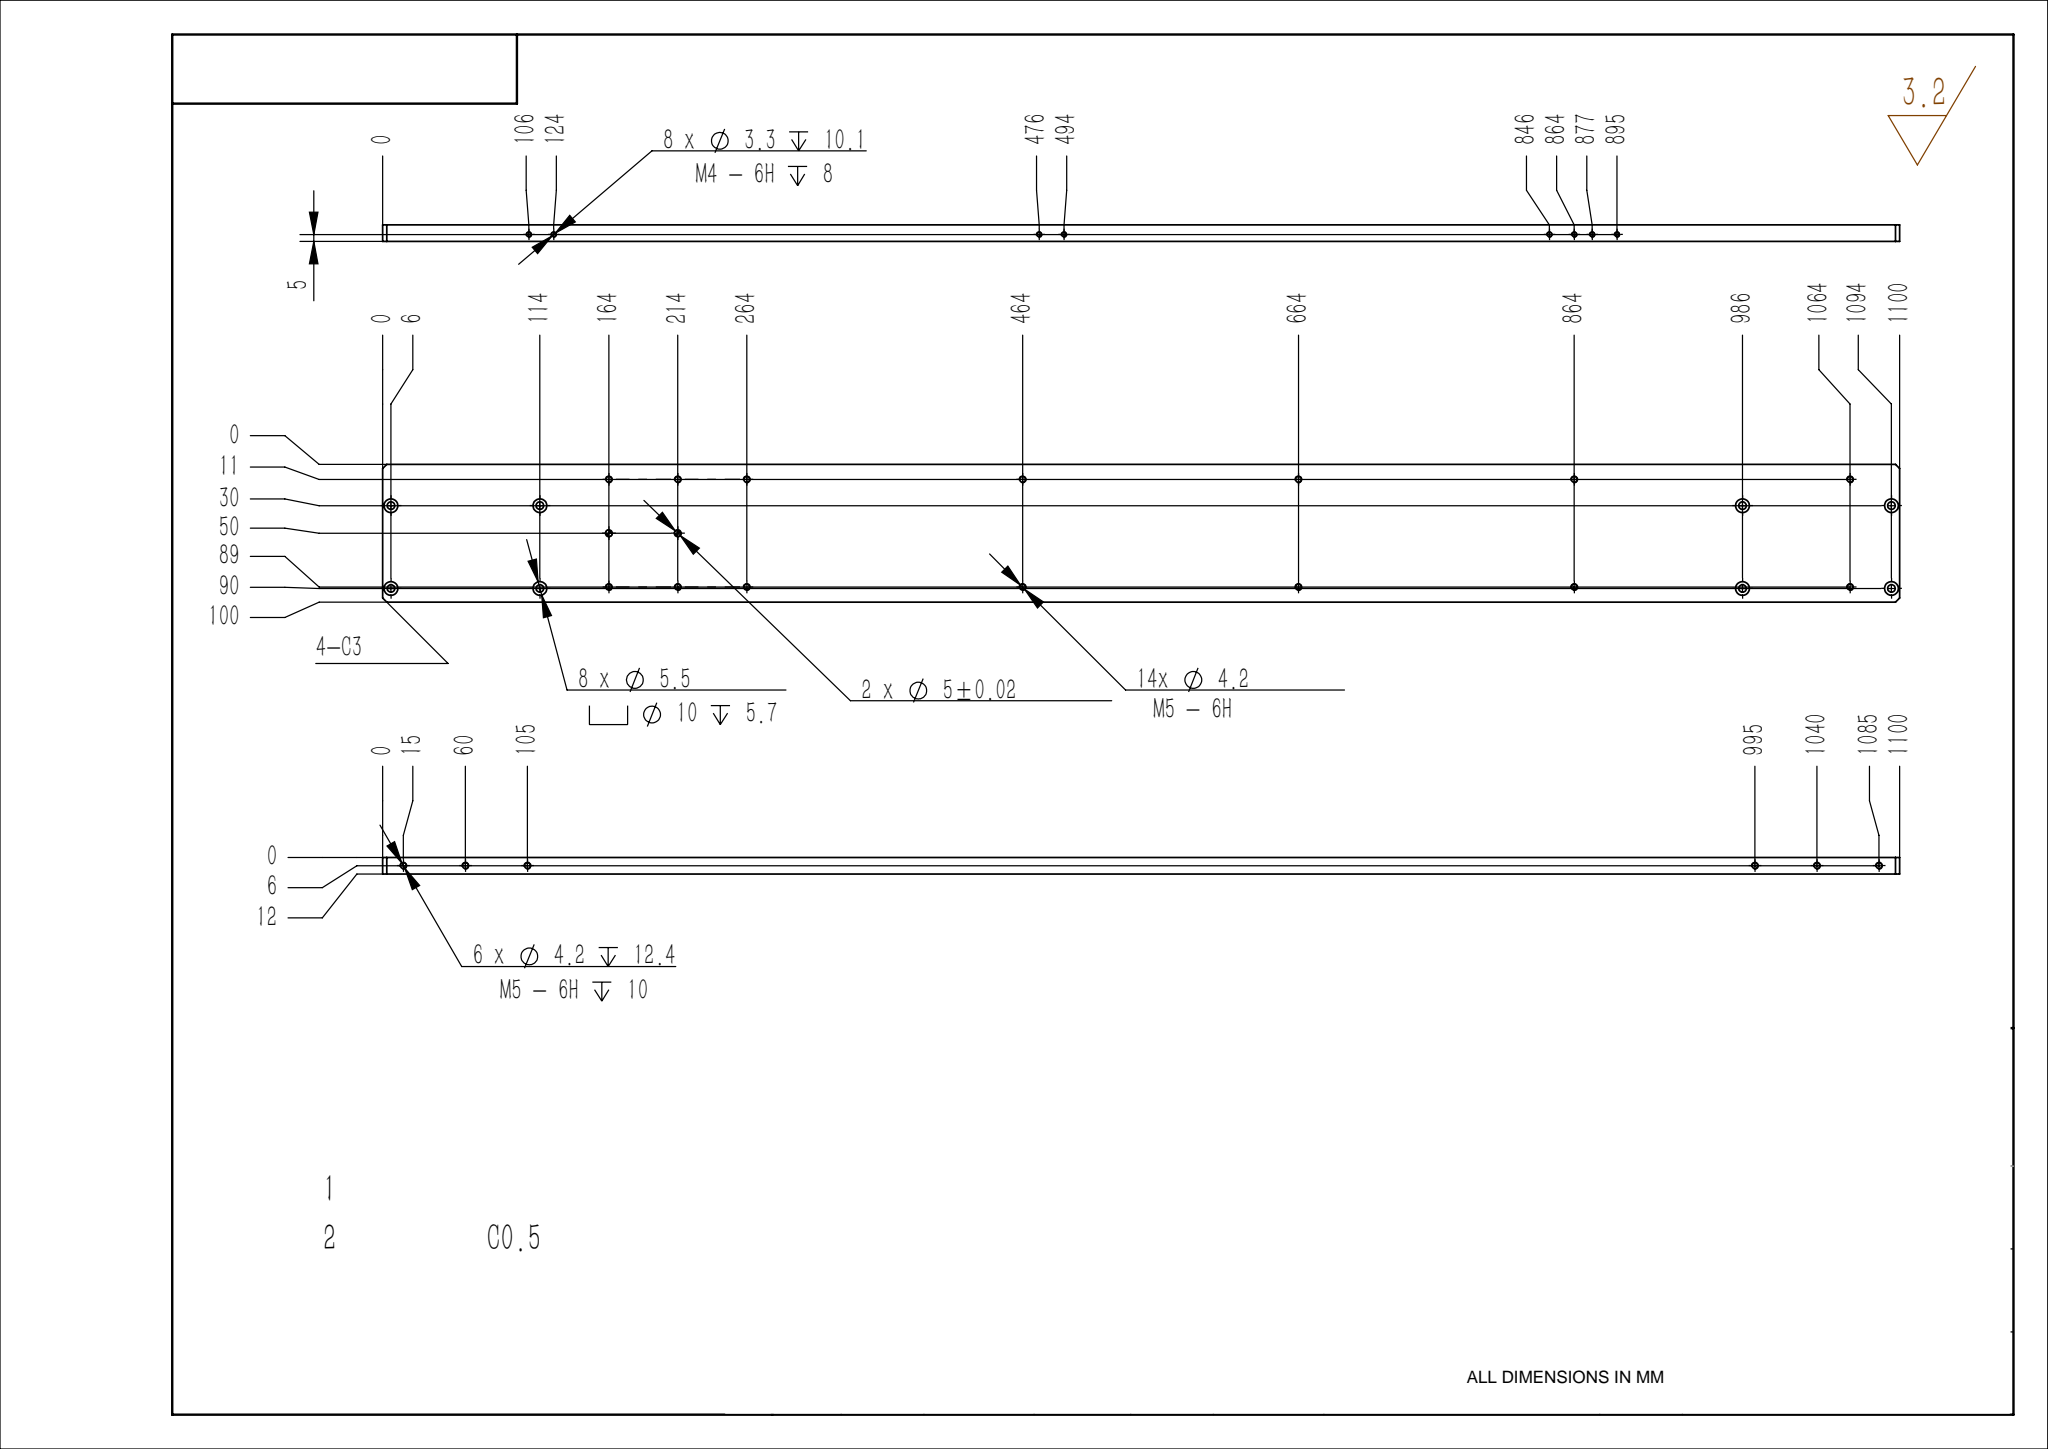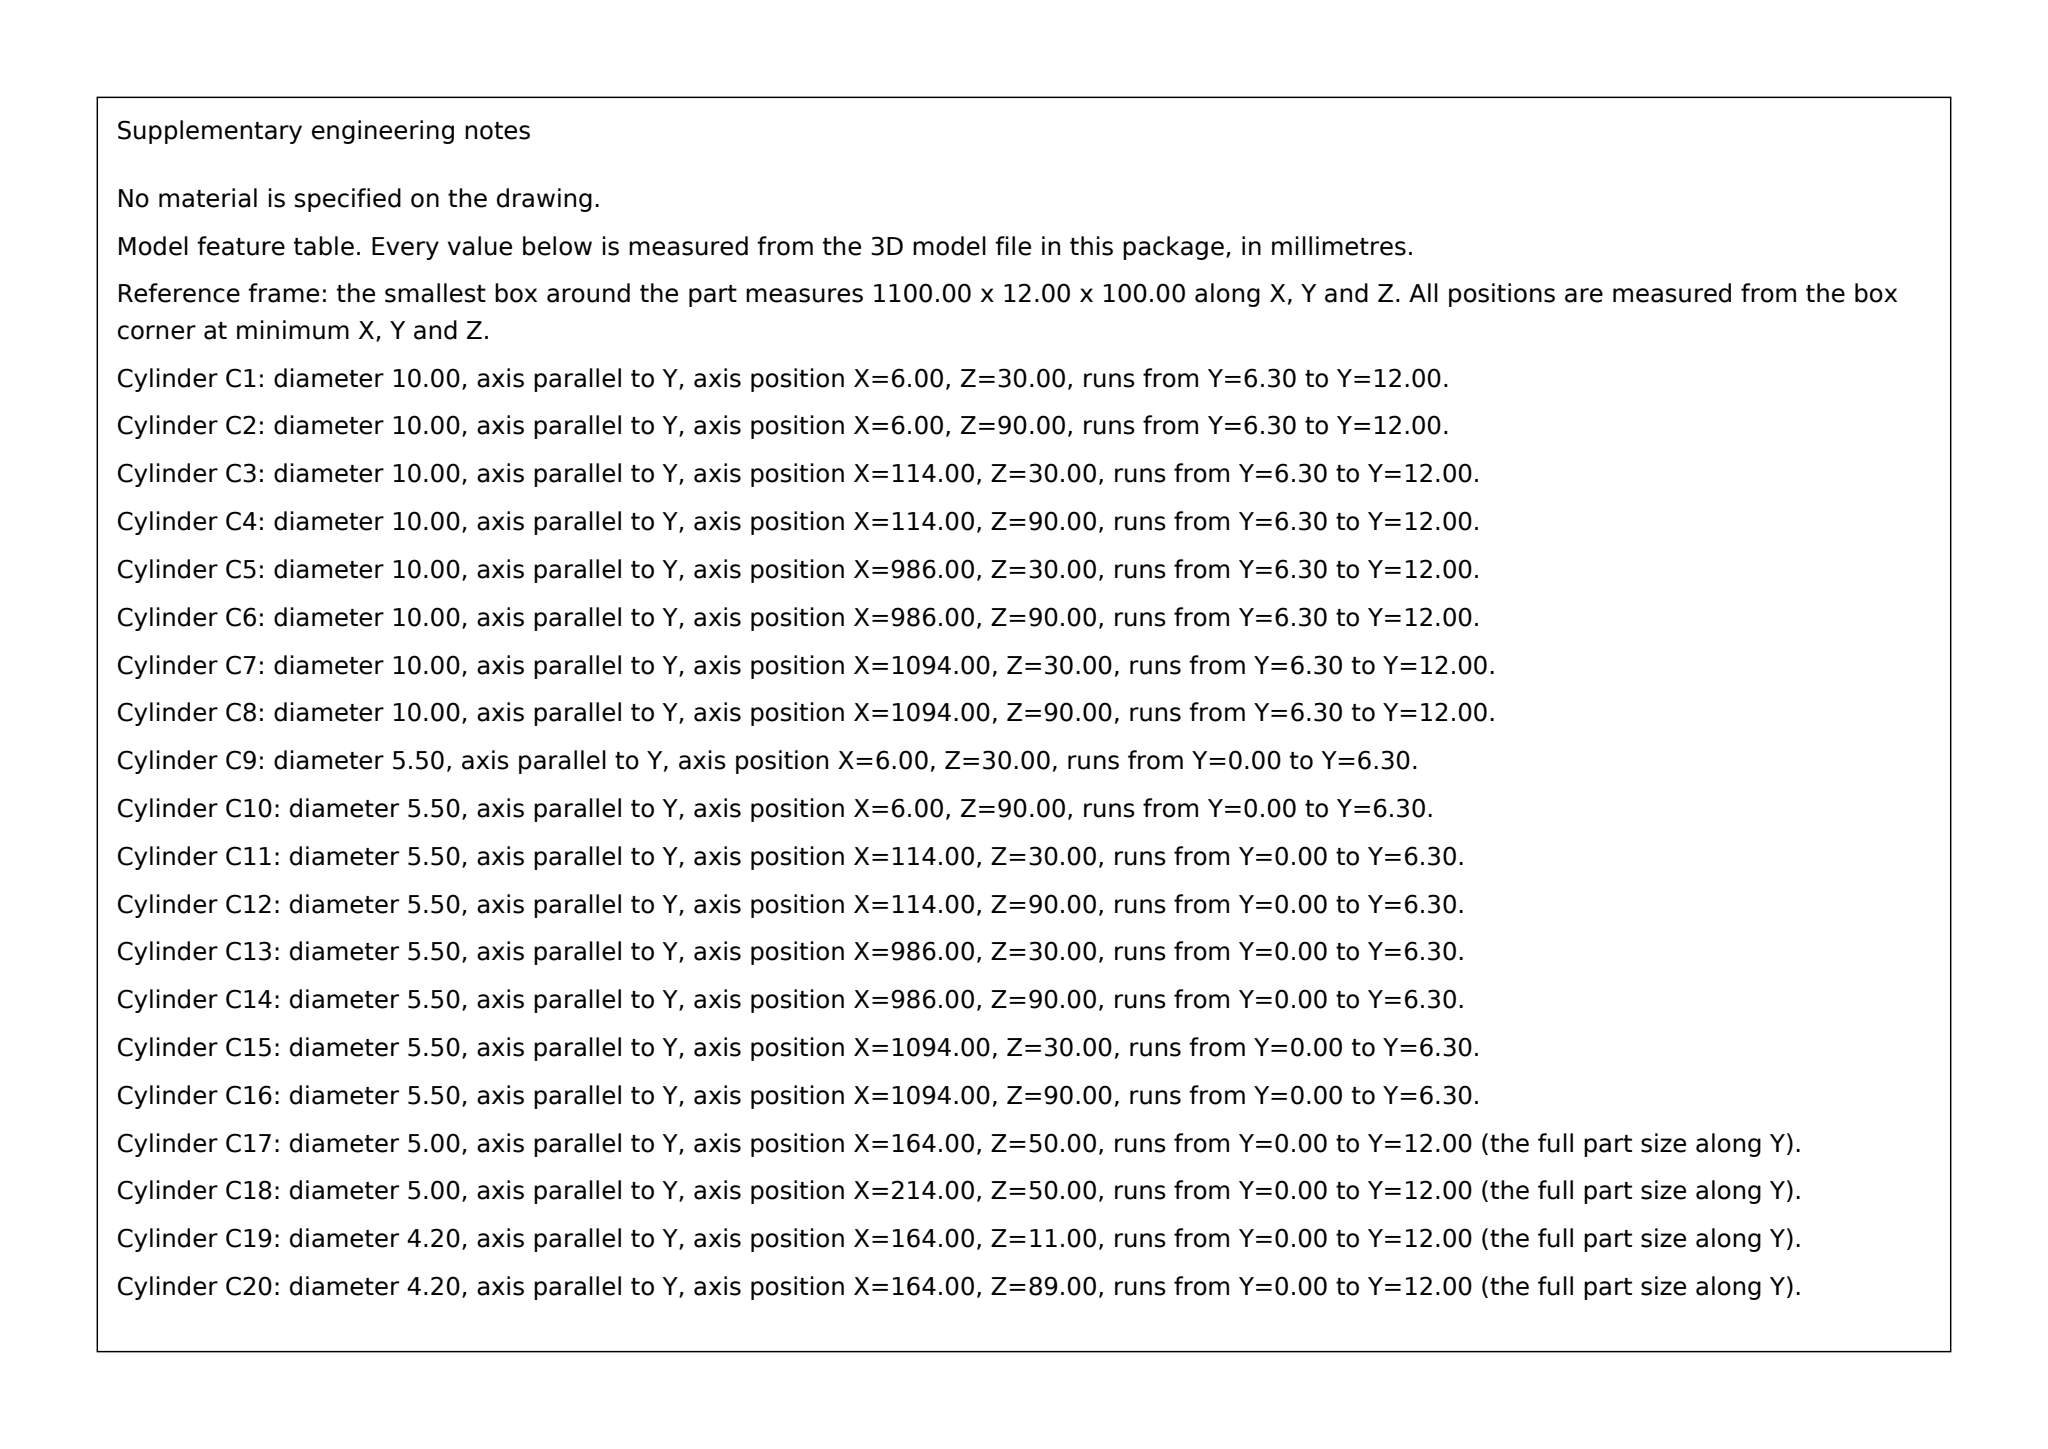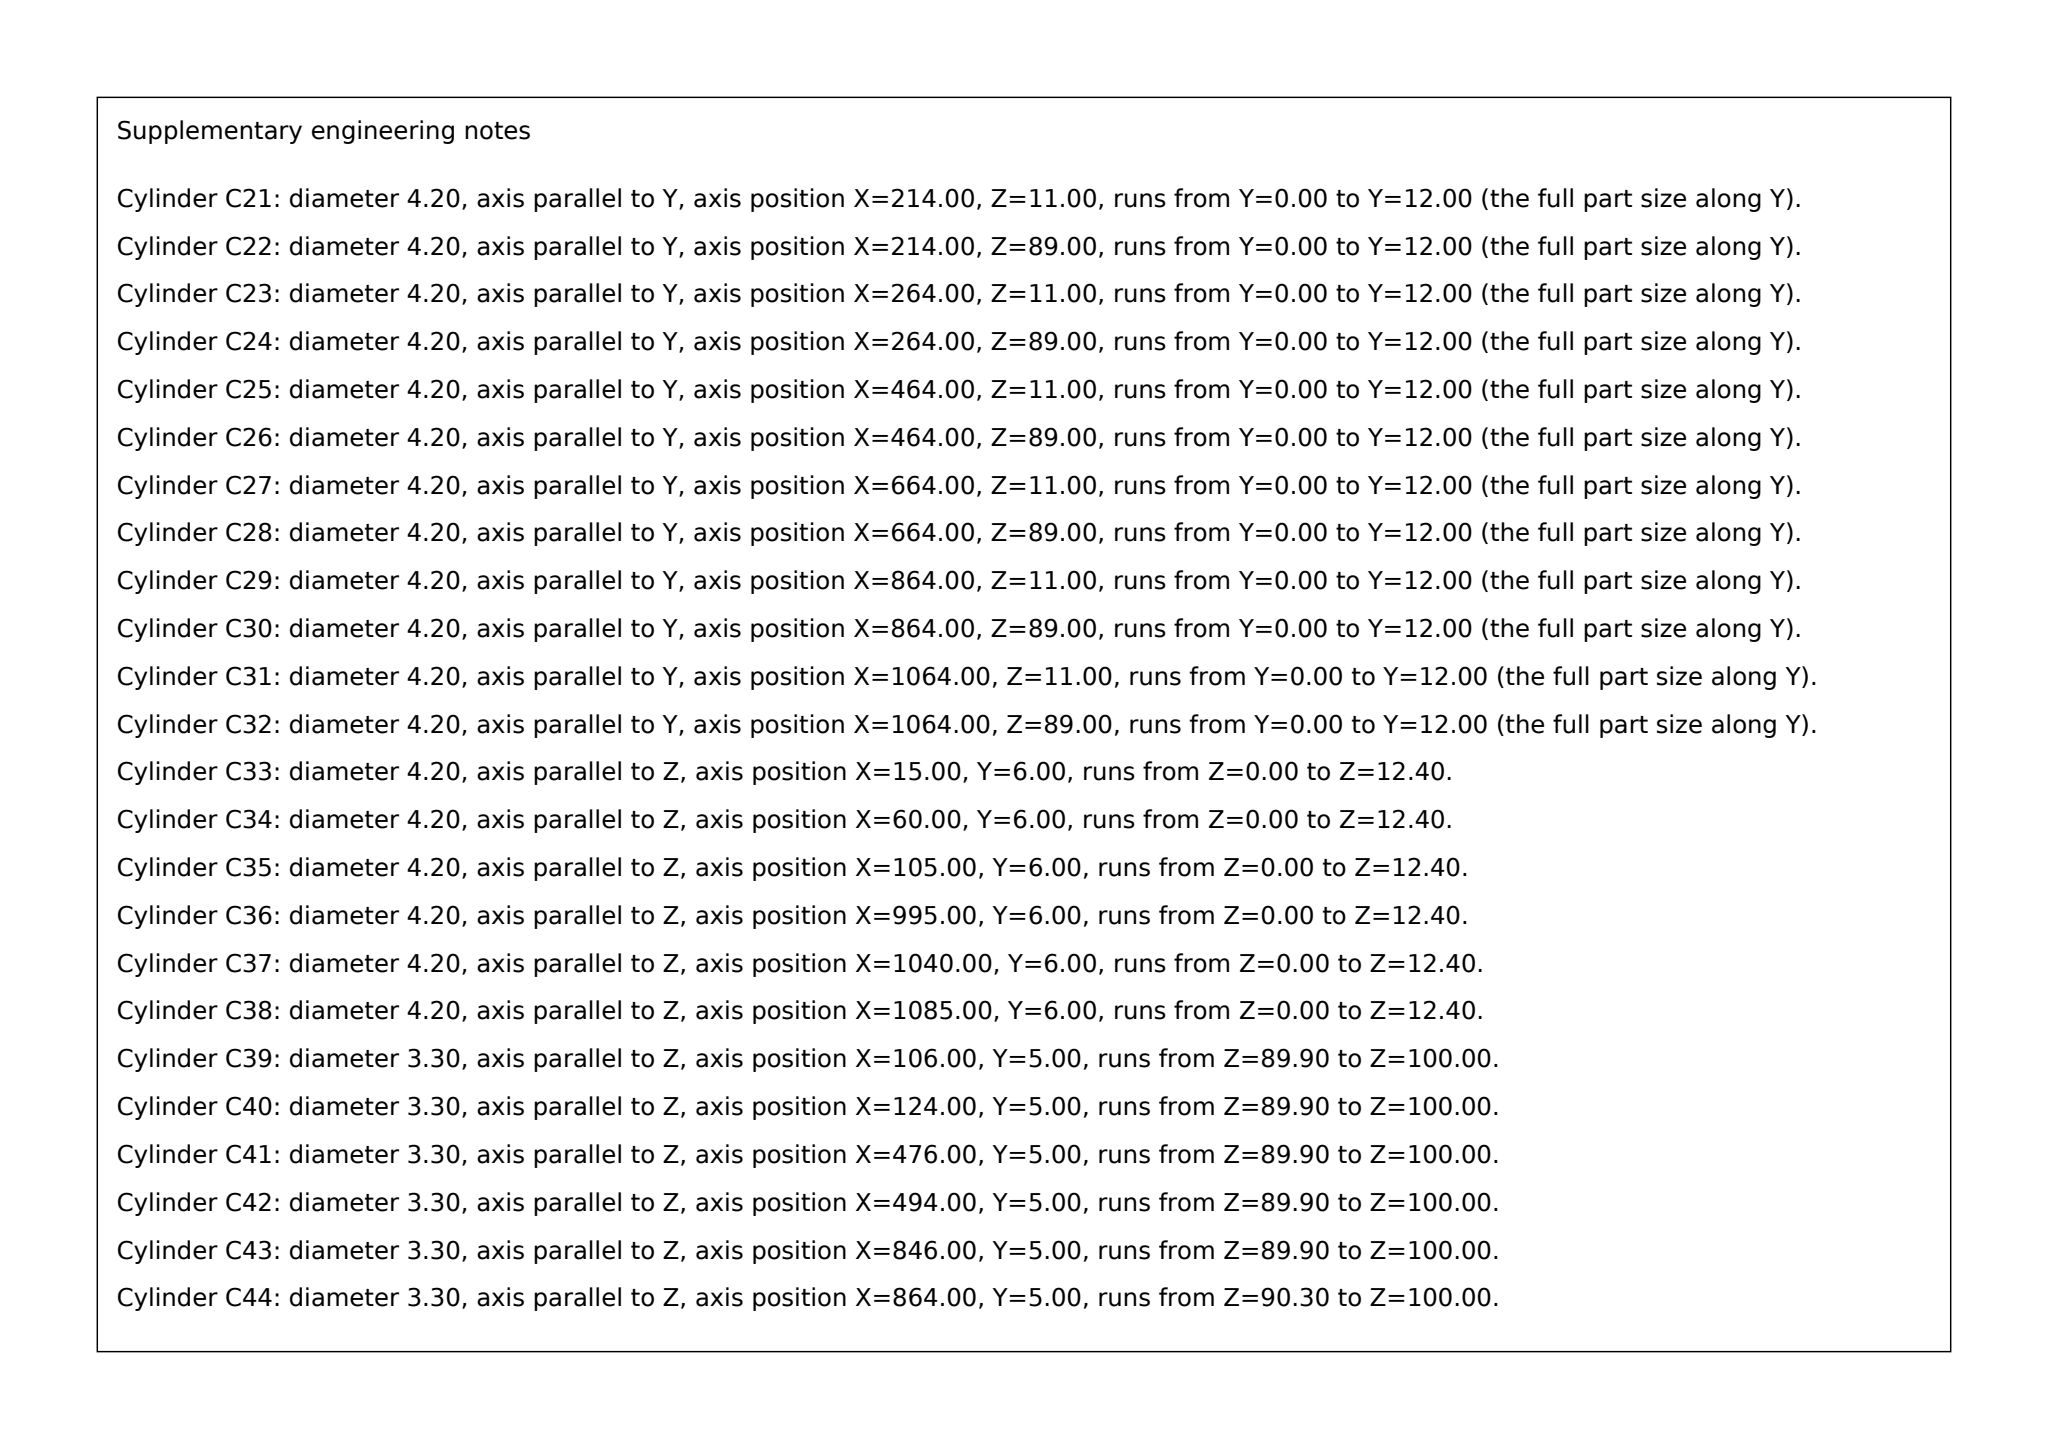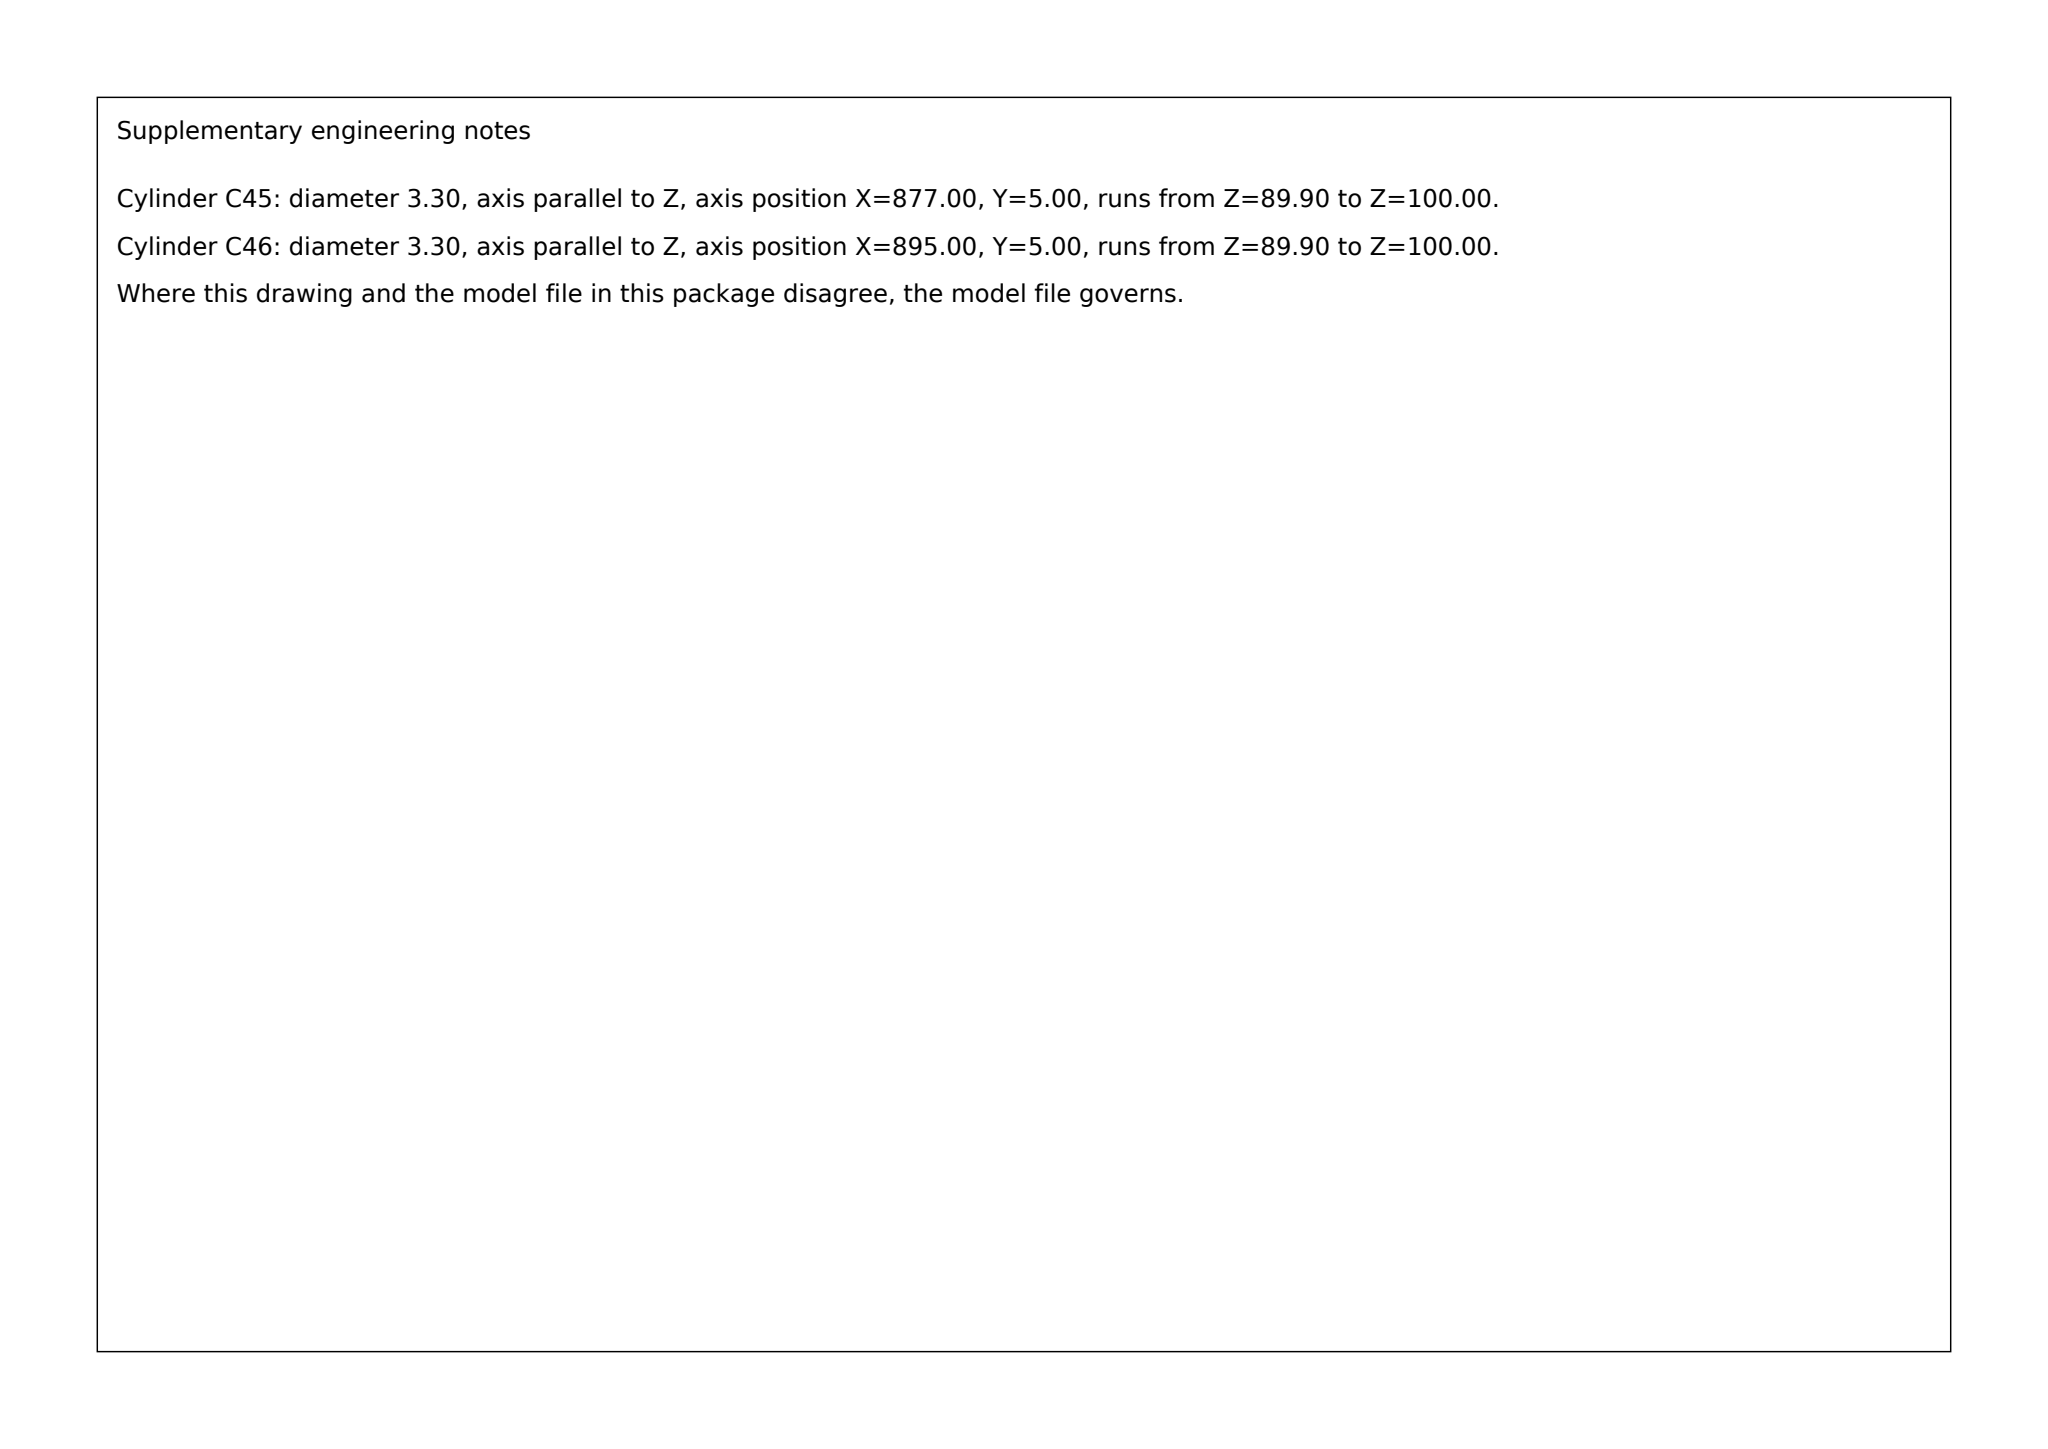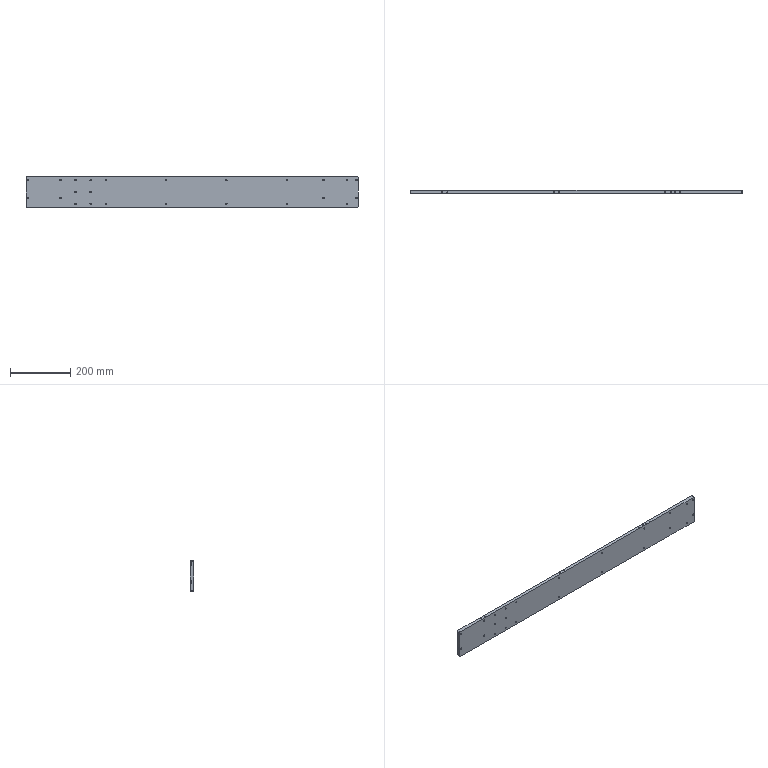Part | SolidWorks | mm | 1 solid | 136 faces | box 1100 x 12 x 100 mm | volume 1310439 mm3 | cylinder 92 | cone 26 | plane 18 | commonest cylinder face diameters 4.2 x40 3.3 x16 10 x16 5.5 x16 5 x4
build123d program:
from build123d import *

# Parameters (mm, degrees)
SKETCH1_W                                         = 1100
SKETCH1_H                                         = 100
BOSS_EXTRUDE1_DEPTH                               = 12
CHAMFER1_SIZE                                     = 3
HOLE_SIZE_ACCORDING_TO_TYPE_1_OF_HEXA_D           = 5.5
HOLE_SIZE_ACCORDING_TO_TYPE_1_OF_HEXA_CBORE_D     = 10
HOLE_SIZE_ACCORDING_TO_TYPE_1_OF_HEXA_CBORE_DEPTH = 5.7
HOLE_SIZE_ACCORDING_TO_TYPE_2_OF_HEXA_D           = 5.5
HOLE_SIZE_ACCORDING_TO_TYPE_2_OF_HEXA_CBORE_D     = 10
HOLE_SIZE_ACCORDING_TO_TYPE_2_OF_HEXA_CBORE_DEPTH = 5.7
M5_TAPPED_HOLE1_D                                 = 4.2
M5_TAPPED_HOLE1_DEPTH                             = 12.4
M5_TAPPED_HOLE1_TIP                               = 1.262
M5_TAPPED_HOLE2_D                                 = 4.2
M5_TAPPED_HOLE3_D                                 = 4.2
LPATTERN1_COUNT                                   = 4
LPATTERN1_PITCH                                   = 200
LPATTERN2_COUNT                                   = 3
LPATTERN2_PITCH                                   = 50
SIZE_MM_DOWEL_PIN_HOLE1_D                         = 5
M4_TAPPED_HOLE1_D                                 = 3.3
M4_TAPPED_HOLE1_DEPTH                             = 10.1
M4_TAPPED_HOLE1_TIP                               = 0.9914


with BuildPart() as part:
    # Sketch1 → Boss-Extrude1 (new body)
    with BuildSketch(Plane(origin=(0, 0, 0), x_dir=(1, 0, 0), z_dir=(0, 1, 0))):
        Rectangle(SKETCH1_W, SKETCH1_H)
    extrude(amount=BOSS_EXTRUDE1_DEPTH)

    # Chamfer1
    chamfer1_edges = [part.edges().sort_by_distance(p)[0] for p in [
        (550, 6, 50),
        (-550, 6, 50),
        (-550, 6, -50),
        (550, 6, -50),
    ]]
    chamfer(chamfer1_edges, length=CHAMFER1_SIZE)

    # Hole Size _ according to_ Type 1 of Hexa (through all)
    with Locations(Plane(origin=(0, 12, 0), x_dir=(1, 0, 0), z_dir=(0, 1, 0))):
        with Locations((-544, -40), (-544, 20), (-436, -40), (-436, 20)):
            CounterBoreHole(HOLE_SIZE_ACCORDING_TO_TYPE_1_OF_HEXA_D / 2, HOLE_SIZE_ACCORDING_TO_TYPE_1_OF_HEXA_CBORE_D / 2, HOLE_SIZE_ACCORDING_TO_TYPE_1_OF_HEXA_CBORE_DEPTH)

    # Hole Size _ according to_ Type 2 of Hexa (through all)
    with Locations(Plane(origin=(0, 12, 0), x_dir=(1, 0, 0), z_dir=(0, 1, 0))):
        with Locations((544, -40), (544, 20), (436, -40), (436, 20)):
            CounterBoreHole(HOLE_SIZE_ACCORDING_TO_TYPE_2_OF_HEXA_D / 2, HOLE_SIZE_ACCORDING_TO_TYPE_2_OF_HEXA_CBORE_D / 2, HOLE_SIZE_ACCORDING_TO_TYPE_2_OF_HEXA_CBORE_DEPTH)

    # M5 Tapped Hole1
    with Locations(Plane(origin=(0, 0, -50), x_dir=(-1, 0, 0), z_dir=(0, 0, -1))):
        with Locations((535, 6), (490, 6), (445, 6), (-445, 6), (-490, 6), (-535, 6)):
            Hole(M5_TAPPED_HOLE1_D / 2, depth=M5_TAPPED_HOLE1_DEPTH)
            with Locations((0, 0, -(M5_TAPPED_HOLE1_DEPTH + M5_TAPPED_HOLE1_TIP / 2))):  # 118° drill point
                Cone(0, M5_TAPPED_HOLE1_D / 2, M5_TAPPED_HOLE1_TIP, mode=Mode.SUBTRACT)

    # M5 Tapped Hole2 (through all)
    with Locations(Plane(origin=(0, 12, 0), x_dir=(1, 0, 0), z_dir=(0, 1, 0))):
        with Locations((-386, -39), (-386, 39)):
            m5_tapped_hole2 = Hole(M5_TAPPED_HOLE2_D / 2)

    # M5 Tapped Hole3 (through all)
    with Locations(Plane(origin=(0, 12, 0), x_dir=(1, 0, 0), z_dir=(0, 1, 0))):
        with Locations((514, -39), (514, 39)):
            m5_tapped_hole3 = Hole(M5_TAPPED_HOLE3_D / 2)

    # LPattern1: M5 Tapped Hole3 ×4
    with Locations(*[(-i * LPATTERN1_PITCH, 0, 0) for i in range(1, LPATTERN1_COUNT)]):
        add(m5_tapped_hole3, mode=Mode.SUBTRACT)

    # LPattern2: M5 Tapped Hole2 ×3
    with Locations(*[(i * LPATTERN2_PITCH, 0, 0) for i in range(1, LPATTERN2_COUNT)]):
        add(m5_tapped_hole2, mode=Mode.SUBTRACT)

    # Size mm Dowel Pin Hole1 (through all)
    with Locations(Plane(origin=(0, 12, 0), x_dir=(1, 0, 0), z_dir=(0, 1, 0))):
        with Locations((-386, 0), (-336, 0)):
            Hole(SIZE_MM_DOWEL_PIN_HOLE1_D / 2)

    # M4 Tapped Hole1
    with Locations(Plane.XY.offset(50)):
        with Locations((345, 5), (327, 5), (314, 5), (296, 5), (-56, 5), (-74, 5), (-426, 5), (-444, 5)):
            Hole(M4_TAPPED_HOLE1_D / 2, depth=M4_TAPPED_HOLE1_DEPTH)
            with Locations((0, 0, -(M4_TAPPED_HOLE1_DEPTH + M4_TAPPED_HOLE1_TIP / 2))):  # 118° drill point
                Cone(0, M4_TAPPED_HOLE1_D / 2, M4_TAPPED_HOLE1_TIP, mode=Mode.SUBTRACT)


solid = part.part